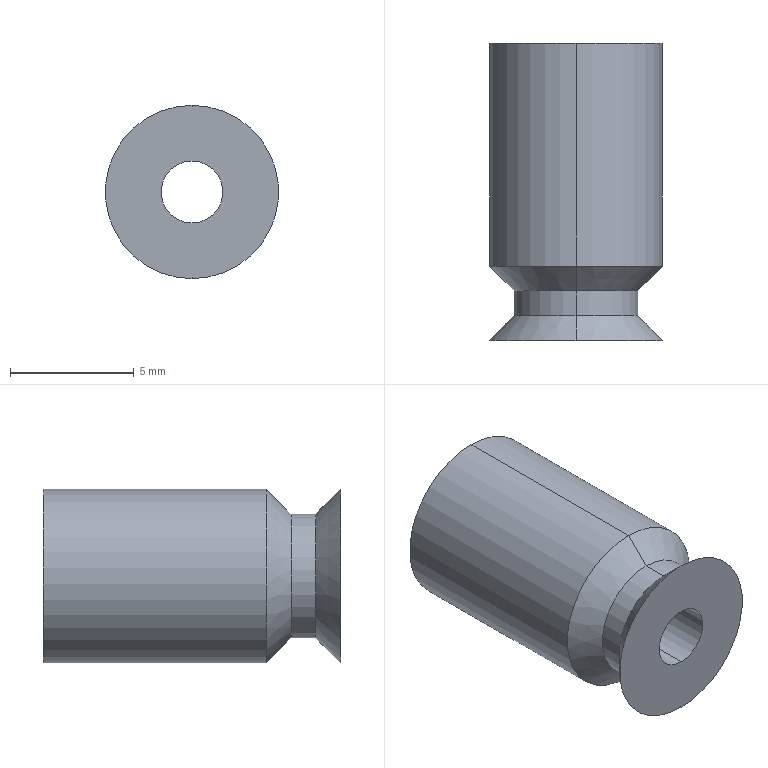Component | SolidWorks | ZPT06UNK6_B5_A80214-1_ZP06U_T_B0214-1 | 1 solid | 12 faces | box 7 x 12 x 7 mm | volume 364 mm3 | cylinder 6 | cone 4 | plane 2 | commonest cylinder face diameters 7 x2 5 x2 2.5 x2
build123d program:
from build123d import *


with BuildPart() as part:
    # Sketch1 → Revolve1 (revolve)
    with BuildSketch(Plane.XY, mode=Mode.PRIVATE) as revolve1_sk:
        Polygon((1.25, 0), (3.5, 0), (2.5, 1), (2.5, 2), (3.5, 3), (3.5, 12), (1.25, 12), align=None)
    revolve(revolve1_sk.sketch.rotate(Axis((0, 0, 0), (0, 1, 0)), 270), axis=Axis((0, 0, 0), (0, 1, 0)))


solid = part.part

# Placed as in the assembly
solid = solid.moved(Location((-75, -83, 9.1), (0, 0, 0)))
STEP:
#1=COLOUR_RGB('',0.7922,0.8196,0.9333);
#2=FILL_AREA_STYLE_COLOUR('',#1);
#3=FILL_AREA_STYLE('',(#2));
#4=SURFACE_STYLE_FILL_AREA(#3);
#5=SURFACE_SIDE_STYLE('',(#4));
#6=SURFACE_STYLE_USAGE(.BOTH.,#5);
#7=PRESENTATION_STYLE_ASSIGNMENT((#6));
#8=CARTESIAN_POINT('',(-2.953,-3.15,0.4961));
#9=VERTEX_POINT('',#8);
#10=CARTESIAN_POINT('',(-2.953,-3.15,0.2205));
#11=VERTEX_POINT('',#10);
#12=CARTESIAN_POINT('',(-2.953,-3.15,0.3583));
#13=DIRECTION('',(0.,1.,0.));
#14=DIRECTION('',(0.,0.,1.));
#15=AXIS2_PLACEMENT_3D('',#12,#13,#14);
#16=CIRCLE('',#15,0.1378);
#17=EDGE_CURVE('',#9,#11,#16,.T.);
#18=ORIENTED_EDGE('',*,*,#17,.T.);
#19=CARTESIAN_POINT('',(-2.953,-2.795,0.2205));
#20=VERTEX_POINT('',#19);
#21=CARTESIAN_POINT('',(-2.953,-3.268,0.2205));
#22=DIRECTION('',(0.,1.,0.));
#23=VECTOR('',#22,39.37);
#24=LINE('',#21,#23);
#25=EDGE_CURVE('',#11,#20,#24,.T.);
#26=ORIENTED_EDGE('',*,*,#25,.T.);
#27=CARTESIAN_POINT('',(-2.953,-2.795,0.4961));
#28=VERTEX_POINT('',#27);
#29=CARTESIAN_POINT('',(-2.953,-2.795,0.3583));
#30=DIRECTION('',(0.,1.,0.));
#31=DIRECTION('',(0.,0.,1.));
#32=AXIS2_PLACEMENT_3D('',#29,#30,#31);
#33=CIRCLE('',#32,0.1378);
#34=EDGE_CURVE('',#28,#20,#33,.T.);
#35=ORIENTED_EDGE('',*,*,#34,.F.);
#36=CARTESIAN_POINT('',(-2.953,-3.268,0.4961));
#37=DIRECTION('',(0.,1.,0.));
#38=VECTOR('',#37,39.37);
#39=LINE('',#36,#38);
#40=EDGE_CURVE('',#9,#28,#39,.T.);
#41=ORIENTED_EDGE('',*,*,#40,.F.);
#42=EDGE_LOOP('',(#18,#26,#35,#41));
#43=FACE_OUTER_BOUND('',#42,.T.);
#44=CARTESIAN_POINT('',(-2.953,-3.268,0.3583));
#45=DIRECTION('',(0.,1.,0.));
#46=DIRECTION('',(0.,0.,1.));
#47=AXIS2_PLACEMENT_3D('',#44,#45,#46);
#48=CYLINDRICAL_SURFACE('',#47,0.1378);
#49=ADVANCED_FACE('',(#43),#48,.T.);
#50=CARTESIAN_POINT('',(-2.953,-3.189,0.4567));
#51=VERTEX_POINT('',#50);
#52=CARTESIAN_POINT('',(-2.953,-3.189,0.2598));
#53=VERTEX_POINT('',#52);
#54=CARTESIAN_POINT('',(-2.953,-3.189,0.3583));
#55=DIRECTION('',(0.,1.,0.));
#56=DIRECTION('',(0.,0.,1.));
#57=AXIS2_PLACEMENT_3D('',#54,#55,#56);
#58=CIRCLE('',#57,0.09843);
#59=EDGE_CURVE('',#51,#53,#58,.T.);
#60=ORIENTED_EDGE('',*,*,#59,.T.);
#61=CARTESIAN_POINT('',(-2.953,-3.189,0.2598));
#62=DIRECTION('',(0.,0.7071,-0.7071));
#63=VECTOR('',#62,39.37);
#64=LINE('',#61,#63);
#65=EDGE_CURVE('',#53,#11,#64,.T.);
#66=ORIENTED_EDGE('',*,*,#65,.T.);
#67=ORIENTED_EDGE('',*,*,#17,.F.);
#68=CARTESIAN_POINT('',(-2.953,-3.189,0.4567));
#69=DIRECTION('',(0.,0.7071,0.7071));
#70=VECTOR('',#69,39.37);
#71=LINE('',#68,#70);
#72=EDGE_CURVE('',#51,#9,#71,.T.);
#73=ORIENTED_EDGE('',*,*,#72,.F.);
#74=EDGE_LOOP('',(#60,#66,#67,#73));
#75=FACE_OUTER_BOUND('',#74,.T.);
#76=CARTESIAN_POINT('',(-2.953,-3.189,0.3583));
#77=DIRECTION('',(0.,1.,0.));
#78=DIRECTION('',(0.,0.,1.));
#79=AXIS2_PLACEMENT_3D('',#76,#77,#78);
#80=CONICAL_SURFACE('',#79,0.09843,0.7854);
#81=ADVANCED_FACE('',(#75),#80,.T.);
#82=CARTESIAN_POINT('',(-2.953,-3.228,0.4567));
#83=VERTEX_POINT('',#82);
#84=CARTESIAN_POINT('',(-2.953,-3.228,0.2598));
#85=VERTEX_POINT('',#84);
#86=CARTESIAN_POINT('',(-2.953,-3.228,0.3583));
#87=DIRECTION('',(0.,1.,0.));
#88=DIRECTION('',(0.,0.,1.));
#89=AXIS2_PLACEMENT_3D('',#86,#87,#88);
#90=CIRCLE('',#89,0.09843);
#91=EDGE_CURVE('',#83,#85,#90,.T.);
#92=ORIENTED_EDGE('',*,*,#91,.T.);
#93=CARTESIAN_POINT('',(-2.953,-3.268,0.2598));
#94=DIRECTION('',(0.,1.,0.));
#95=VECTOR('',#94,39.37);
#96=LINE('',#93,#95);
#97=EDGE_CURVE('',#85,#53,#96,.T.);
#98=ORIENTED_EDGE('',*,*,#97,.T.);
#99=ORIENTED_EDGE('',*,*,#59,.F.);
#100=CARTESIAN_POINT('',(-2.953,-3.268,0.4567));
#101=DIRECTION('',(0.,1.,0.));
#102=VECTOR('',#101,39.37);
#103=LINE('',#100,#102);
#104=EDGE_CURVE('',#83,#51,#103,.T.);
#105=ORIENTED_EDGE('',*,*,#104,.F.);
#106=EDGE_LOOP('',(#92,#98,#99,#105));
#107=FACE_OUTER_BOUND('',#106,.T.);
#108=CARTESIAN_POINT('',(-2.953,-3.268,0.3583));
#109=DIRECTION('',(0.,1.,0.));
#110=DIRECTION('',(0.,0.,1.));
#111=AXIS2_PLACEMENT_3D('',#108,#109,#110);
#112=CYLINDRICAL_SURFACE('',#111,0.09843);
#113=ADVANCED_FACE('',(#107),#112,.T.);
#114=ORIENTED_EDGE('',*,*,#91,.F.);
#115=CARTESIAN_POINT('',(-2.953,-3.268,0.4961));
#116=VERTEX_POINT('',#115);
#117=CARTESIAN_POINT('',(-2.953,-3.268,0.4961));
#118=DIRECTION('',(0.,-0.7071,0.7071));
#119=VECTOR('',#118,39.37);
#120=LINE('',#117,#119);
#121=EDGE_CURVE('',#83,#116,#120,.T.);
#122=ORIENTED_EDGE('',*,*,#121,.T.);
#123=CARTESIAN_POINT('',(-2.953,-3.268,0.2205));
#124=VERTEX_POINT('',#123);
#125=CARTESIAN_POINT('',(-2.953,-3.268,0.3583));
#126=DIRECTION('',(0.,1.,0.));
#127=DIRECTION('',(0.,0.,1.));
#128=AXIS2_PLACEMENT_3D('',#125,#126,#127);
#129=CIRCLE('',#128,0.1378);
#130=EDGE_CURVE('',#116,#124,#129,.T.);
#131=ORIENTED_EDGE('',*,*,#130,.T.);
#132=CARTESIAN_POINT('',(-2.953,-3.268,0.2205));
#133=DIRECTION('',(0.,-0.7071,-0.7071));
#134=VECTOR('',#133,39.37);
#135=LINE('',#132,#134);
#136=EDGE_CURVE('',#85,#124,#135,.T.);
#137=ORIENTED_EDGE('',*,*,#136,.F.);
#138=EDGE_LOOP('',(#114,#122,#131,#137));
#139=FACE_OUTER_BOUND('',#138,.T.);
#140=CARTESIAN_POINT('',(-2.953,-3.268,0.3583));
#141=DIRECTION('',(0.,-1.,0.));
#142=DIRECTION('',(0.,0.,-1.));
#143=AXIS2_PLACEMENT_3D('',#140,#141,#142);
#144=CONICAL_SURFACE('',#143,0.1378,0.7854);
#145=ADVANCED_FACE('',(#139),#144,.T.);
#146=CARTESIAN_POINT('',(-2.953,-3.268,0.3091));
#147=VERTEX_POINT('',#146);
#148=CARTESIAN_POINT('',(-2.953,-3.268,0.4075));
#149=VERTEX_POINT('',#148);
#150=CARTESIAN_POINT('',(-2.953,-3.268,0.3583));
#151=DIRECTION('',(0.,1.,0.));
#152=DIRECTION('',(0.,0.,1.));
#153=AXIS2_PLACEMENT_3D('',#150,#151,#152);
#154=CIRCLE('',#153,0.04921);
#155=EDGE_CURVE('',#147,#149,#154,.T.);
#156=ORIENTED_EDGE('',*,*,#155,.F.);
#157=CARTESIAN_POINT('',(-2.953,-2.795,0.3091));
#158=VERTEX_POINT('',#157);
#159=CARTESIAN_POINT('',(-2.953,-3.268,0.3091));
#160=DIRECTION('',(0.,1.,0.));
#161=VECTOR('',#160,39.37);
#162=LINE('',#159,#161);
#163=EDGE_CURVE('',#147,#158,#162,.T.);
#164=ORIENTED_EDGE('',*,*,#163,.T.);
#165=CARTESIAN_POINT('',(-2.953,-2.795,0.4075));
#166=VERTEX_POINT('',#165);
#167=CARTESIAN_POINT('',(-2.953,-2.795,0.3583));
#168=DIRECTION('',(0.,1.,0.));
#169=DIRECTION('',(0.,0.,1.));
#170=AXIS2_PLACEMENT_3D('',#167,#168,#169);
#171=CIRCLE('',#170,0.04921);
#172=EDGE_CURVE('',#158,#166,#171,.T.);
#173=ORIENTED_EDGE('',*,*,#172,.T.);
#174=CARTESIAN_POINT('',(-2.953,-3.268,0.4075));
#175=DIRECTION('',(0.,1.,0.));
#176=VECTOR('',#175,39.37);
#177=LINE('',#174,#176);
#178=EDGE_CURVE('',#149,#166,#177,.T.);
#179=ORIENTED_EDGE('',*,*,#178,.F.);
#180=EDGE_LOOP('',(#156,#164,#173,#179));
#181=FACE_OUTER_BOUND('',#180,.T.);
#182=CARTESIAN_POINT('',(-2.953,-3.268,0.3583));
#183=DIRECTION('',(0.,1.,0.));
#184=DIRECTION('',(0.,0.,1.));
#185=AXIS2_PLACEMENT_3D('',#182,#183,#184);
#186=CYLINDRICAL_SURFACE('',#185,0.04921);
#187=ADVANCED_FACE('',(#181),#186,.F.);
#188=ORIENTED_EDGE('',*,*,#163,.F.);
#189=CARTESIAN_POINT('',(-2.953,-3.268,0.3583));
#190=DIRECTION('',(0.,1.,0.));
#191=DIRECTION('',(0.,0.,1.));
#192=AXIS2_PLACEMENT_3D('',#189,#190,#191);
#193=CIRCLE('',#192,0.04921);
#194=EDGE_CURVE('',#149,#147,#193,.T.);
#195=ORIENTED_EDGE('',*,*,#194,.F.);
#196=ORIENTED_EDGE('',*,*,#178,.T.);
#197=CARTESIAN_POINT('',(-2.953,-2.795,0.3583));
#198=DIRECTION('',(0.,1.,0.));
#199=DIRECTION('',(0.,0.,1.));
#200=AXIS2_PLACEMENT_3D('',#197,#198,#199);
#201=CIRCLE('',#200,0.04921);
#202=EDGE_CURVE('',#166,#158,#201,.T.);
#203=ORIENTED_EDGE('',*,*,#202,.T.);
#204=EDGE_LOOP('',(#188,#195,#196,#203));
#205=FACE_OUTER_BOUND('',#204,.T.);
#206=CARTESIAN_POINT('',(-2.953,-3.268,0.3583));
#207=DIRECTION('',(0.,1.,0.));
#208=DIRECTION('',(0.,0.,1.));
#209=AXIS2_PLACEMENT_3D('',#206,#207,#208);
#210=CYLINDRICAL_SURFACE('',#209,0.04921);
#211=ADVANCED_FACE('',(#205),#210,.F.);
#212=CARTESIAN_POINT('',(-2.953,-3.268,0.3583));
#213=DIRECTION('',(0.,1.,0.));
#214=DIRECTION('',(0.,0.,1.));
#215=AXIS2_PLACEMENT_3D('',#212,#213,#214);
#216=CIRCLE('',#215,0.1378);
#217=EDGE_CURVE('',#124,#116,#216,.T.);
#218=ORIENTED_EDGE('',*,*,#217,.F.);
#219=ORIENTED_EDGE('',*,*,#130,.F.);
#220=EDGE_LOOP('',(#218,#219));
#221=FACE_OUTER_BOUND('',#220,.T.);
#222=ORIENTED_EDGE('',*,*,#194,.T.);
#223=ORIENTED_EDGE('',*,*,#155,.T.);
#224=EDGE_LOOP('',(#222,#223));
#225=FACE_BOUND('',#224,.T.);
#226=CARTESIAN_POINT('',(-2.904,-3.268,0.3583));
#227=DIRECTION('',(0.,1.,0.));
#228=DIRECTION('',(0.,0.,1.));
#229=AXIS2_PLACEMENT_3D('',#226,#227,#228);
#230=PLANE('',#229);
#231=ADVANCED_FACE('',(#221,#225),#230,.F.);
#232=ORIENTED_EDGE('',*,*,#121,.F.);
#233=CARTESIAN_POINT('',(-2.953,-3.228,0.3583));
#234=DIRECTION('',(0.,1.,0.));
#235=DIRECTION('',(0.,0.,1.));
#236=AXIS2_PLACEMENT_3D('',#233,#234,#235);
#237=CIRCLE('',#236,0.09843);
#238=EDGE_CURVE('',#85,#83,#237,.T.);
#239=ORIENTED_EDGE('',*,*,#238,.F.);
#240=ORIENTED_EDGE('',*,*,#136,.T.);
#241=ORIENTED_EDGE('',*,*,#217,.T.);
#242=EDGE_LOOP('',(#232,#239,#240,#241));
#243=FACE_OUTER_BOUND('',#242,.T.);
#244=CARTESIAN_POINT('',(-2.953,-3.268,0.3583));
#245=DIRECTION('',(0.,-1.,0.));
#246=DIRECTION('',(0.,0.,-1.));
#247=AXIS2_PLACEMENT_3D('',#244,#245,#246);
#248=CONICAL_SURFACE('',#247,0.1378,0.7854);
#249=ADVANCED_FACE('',(#243),#248,.T.);
#250=ORIENTED_EDGE('',*,*,#97,.F.);
#251=ORIENTED_EDGE('',*,*,#238,.T.);
#252=ORIENTED_EDGE('',*,*,#104,.T.);
#253=CARTESIAN_POINT('',(-2.953,-3.189,0.3583));
#254=DIRECTION('',(0.,1.,0.));
#255=DIRECTION('',(0.,0.,1.));
#256=AXIS2_PLACEMENT_3D('',#253,#254,#255);
#257=CIRCLE('',#256,0.09843);
#258=EDGE_CURVE('',#53,#51,#257,.T.);
#259=ORIENTED_EDGE('',*,*,#258,.F.);
#260=EDGE_LOOP('',(#250,#251,#252,#259));
#261=FACE_OUTER_BOUND('',#260,.T.);
#262=CARTESIAN_POINT('',(-2.953,-3.268,0.3583));
#263=DIRECTION('',(0.,1.,0.));
#264=DIRECTION('',(0.,0.,1.));
#265=AXIS2_PLACEMENT_3D('',#262,#263,#264);
#266=CYLINDRICAL_SURFACE('',#265,0.09843);
#267=ADVANCED_FACE('',(#261),#266,.T.);
#268=ORIENTED_EDGE('',*,*,#65,.F.);
#269=ORIENTED_EDGE('',*,*,#258,.T.);
#270=ORIENTED_EDGE('',*,*,#72,.T.);
#271=CARTESIAN_POINT('',(-2.953,-3.15,0.3583));
#272=DIRECTION('',(0.,1.,0.));
#273=DIRECTION('',(0.,0.,1.));
#274=AXIS2_PLACEMENT_3D('',#271,#272,#273);
#275=CIRCLE('',#274,0.1378);
#276=EDGE_CURVE('',#11,#9,#275,.T.);
#277=ORIENTED_EDGE('',*,*,#276,.F.);
#278=EDGE_LOOP('',(#268,#269,#270,#277));
#279=FACE_OUTER_BOUND('',#278,.T.);
#280=CARTESIAN_POINT('',(-2.953,-3.189,0.3583));
#281=DIRECTION('',(0.,1.,0.));
#282=DIRECTION('',(0.,0.,1.));
#283=AXIS2_PLACEMENT_3D('',#280,#281,#282);
#284=CONICAL_SURFACE('',#283,0.09843,0.7854);
#285=ADVANCED_FACE('',(#279),#284,.T.);
#286=ORIENTED_EDGE('',*,*,#25,.F.);
#287=ORIENTED_EDGE('',*,*,#276,.T.);
#288=ORIENTED_EDGE('',*,*,#40,.T.);
#289=CARTESIAN_POINT('',(-2.953,-2.795,0.3583));
#290=DIRECTION('',(0.,1.,0.));
#291=DIRECTION('',(0.,0.,1.));
#292=AXIS2_PLACEMENT_3D('',#289,#290,#291);
#293=CIRCLE('',#292,0.1378);
#294=EDGE_CURVE('',#20,#28,#293,.T.);
#295=ORIENTED_EDGE('',*,*,#294,.F.);
#296=EDGE_LOOP('',(#286,#287,#288,#295));
#297=FACE_OUTER_BOUND('',#296,.T.);
#298=CARTESIAN_POINT('',(-2.953,-3.268,0.3583));
#299=DIRECTION('',(0.,1.,0.));
#300=DIRECTION('',(0.,0.,1.));
#301=AXIS2_PLACEMENT_3D('',#298,#299,#300);
#302=CYLINDRICAL_SURFACE('',#301,0.1378);
#303=ADVANCED_FACE('',(#297),#302,.T.);
#304=ORIENTED_EDGE('',*,*,#202,.F.);
#305=ORIENTED_EDGE('',*,*,#172,.F.);
#306=EDGE_LOOP('',(#304,#305));
#307=FACE_BOUND('',#306,.T.);
#308=ORIENTED_EDGE('',*,*,#34,.T.);
#309=ORIENTED_EDGE('',*,*,#294,.T.);
#310=EDGE_LOOP('',(#308,#309));
#311=FACE_OUTER_BOUND('',#310,.T.);
#312=CARTESIAN_POINT('',(-2.815,-2.795,0.3583));
#313=DIRECTION('',(0.,-1.,0.));
#314=DIRECTION('',(0.,0.,-1.));
#315=AXIS2_PLACEMENT_3D('',#312,#313,#314);
#316=PLANE('',#315);
#317=ADVANCED_FACE('',(#307,#311),#316,.F.);
#318=CLOSED_SHELL('',(#49,#81,#113,#145,#187,#211,#231,#249,#267,#285,#303,#317));
#319=MANIFOLD_SOLID_BREP('',#318);
#320=STYLED_ITEM('',(#7),#319);
#321=PRESENTATION_LAYER_ASSIGNMENT('','',(#320));
#322=CARTESIAN_POINT('',(0.,0.,0.));
#323=DIRECTION('',(0.,0.,1.));
#324=DIRECTION('',(1.,0.,0.));
#325=AXIS2_PLACEMENT_3D('',#322,#323,#324);
#326=(LENGTH_UNIT()NAMED_UNIT(*)SI_UNIT($,.METRE.));
#327=LENGTH_MEASURE_WITH_UNIT(LENGTH_MEASURE(0.0254),#326);
#328=DIMENSIONAL_EXPONENTS(1.,0.,0.,0.,0.,0.,0.);
#329=(CONVERSION_BASED_UNIT('',#327)LENGTH_UNIT()NAMED_UNIT(#328));
#330=UNCERTAINTY_MEASURE_WITH_UNIT(LENGTH_MEASURE(0.00001),#329,'','');
#331=(NAMED_UNIT(*)PLANE_ANGLE_UNIT()SI_UNIT($,.RADIAN.));
#332=(NAMED_UNIT(*)SI_UNIT($,.STERADIAN.)SOLID_ANGLE_UNIT());
#333=(GEOMETRIC_REPRESENTATION_CONTEXT(3)GLOBAL_UNCERTAINTY_ASSIGNED_CONTEXT((#330))GLOBAL_UNIT_ASSIGNED_CONTEXT((#329,#331,#332))REPRESENTATION_CONTEXT('',''));
#334=ADVANCED_BREP_SHAPE_REPRESENTATION('',(#319,#325),#333);
#335=(LENGTH_UNIT()NAMED_UNIT(*)SI_UNIT($,.METRE.));
#336=LENGTH_MEASURE_WITH_UNIT(LENGTH_MEASURE(0.0254),#335);
#337=DIMENSIONAL_EXPONENTS(1.,0.,0.,0.,0.,0.,0.);
#338=(CONVERSION_BASED_UNIT('',#336)LENGTH_UNIT()NAMED_UNIT(#337));
#339=UNCERTAINTY_MEASURE_WITH_UNIT(LENGTH_MEASURE(0.00001),#338,'','');
#340=(NAMED_UNIT(*)PLANE_ANGLE_UNIT()SI_UNIT($,.RADIAN.));
#341=(NAMED_UNIT(*)SI_UNIT($,.STERADIAN.)SOLID_ANGLE_UNIT());
#342=(GEOMETRIC_REPRESENTATION_CONTEXT(3)GLOBAL_UNCERTAINTY_ASSIGNED_CONTEXT((#339))GLOBAL_UNIT_ASSIGNED_CONTEXT((#338,#340,#341))REPRESENTATION_CONTEXT('',''));
#343=MECHANICAL_DESIGN_GEOMETRIC_PRESENTATION_REPRESENTATION('',(#320),#342);